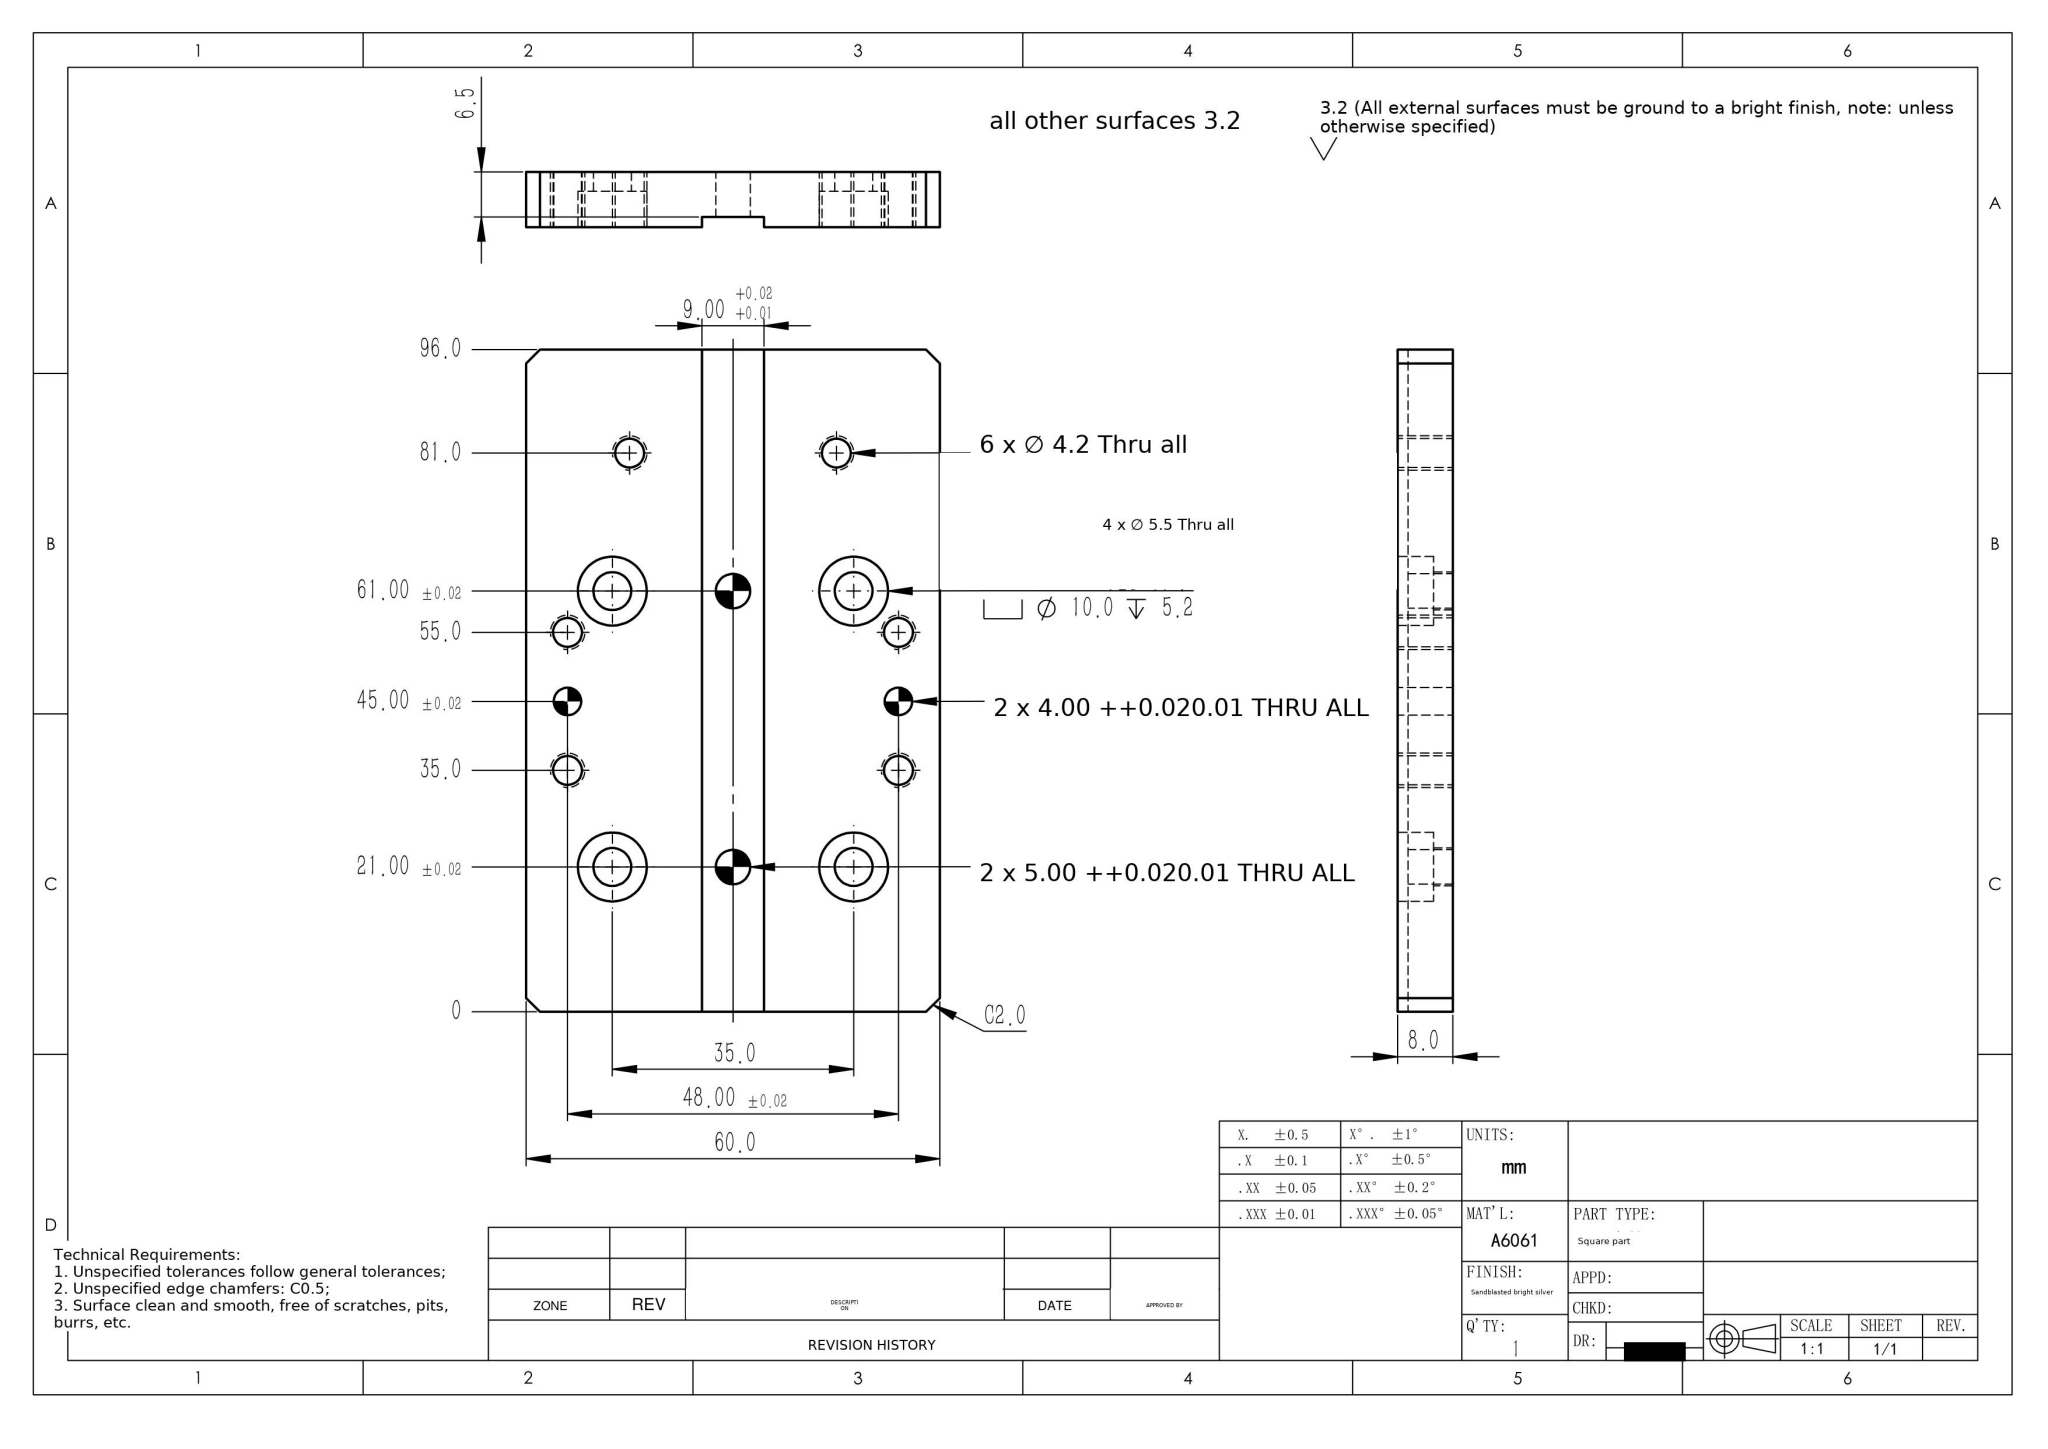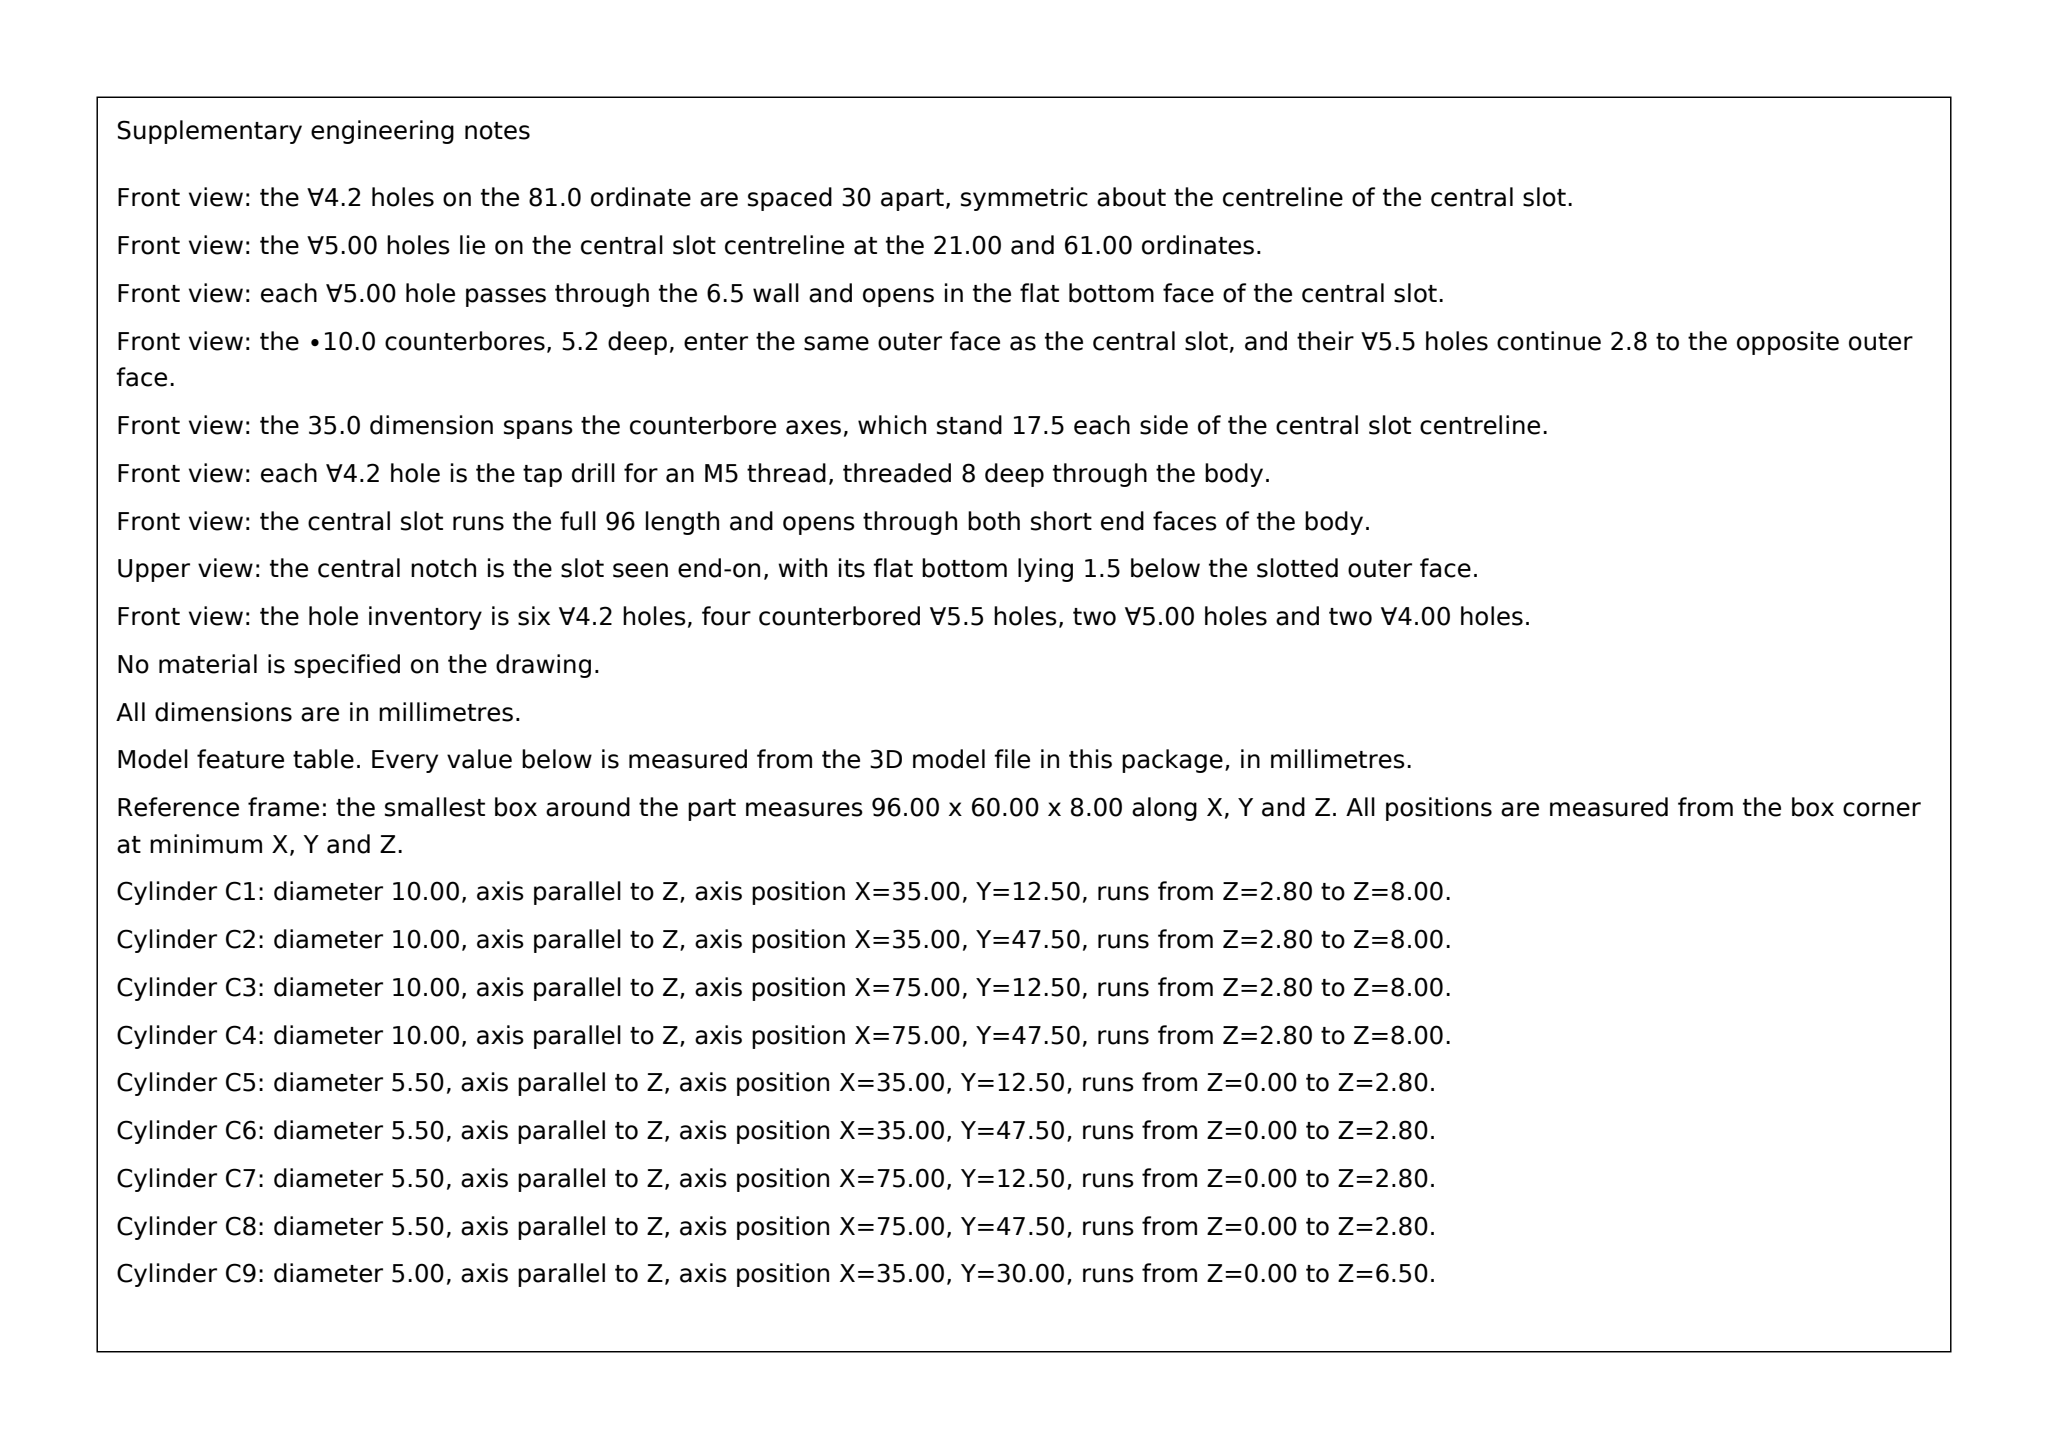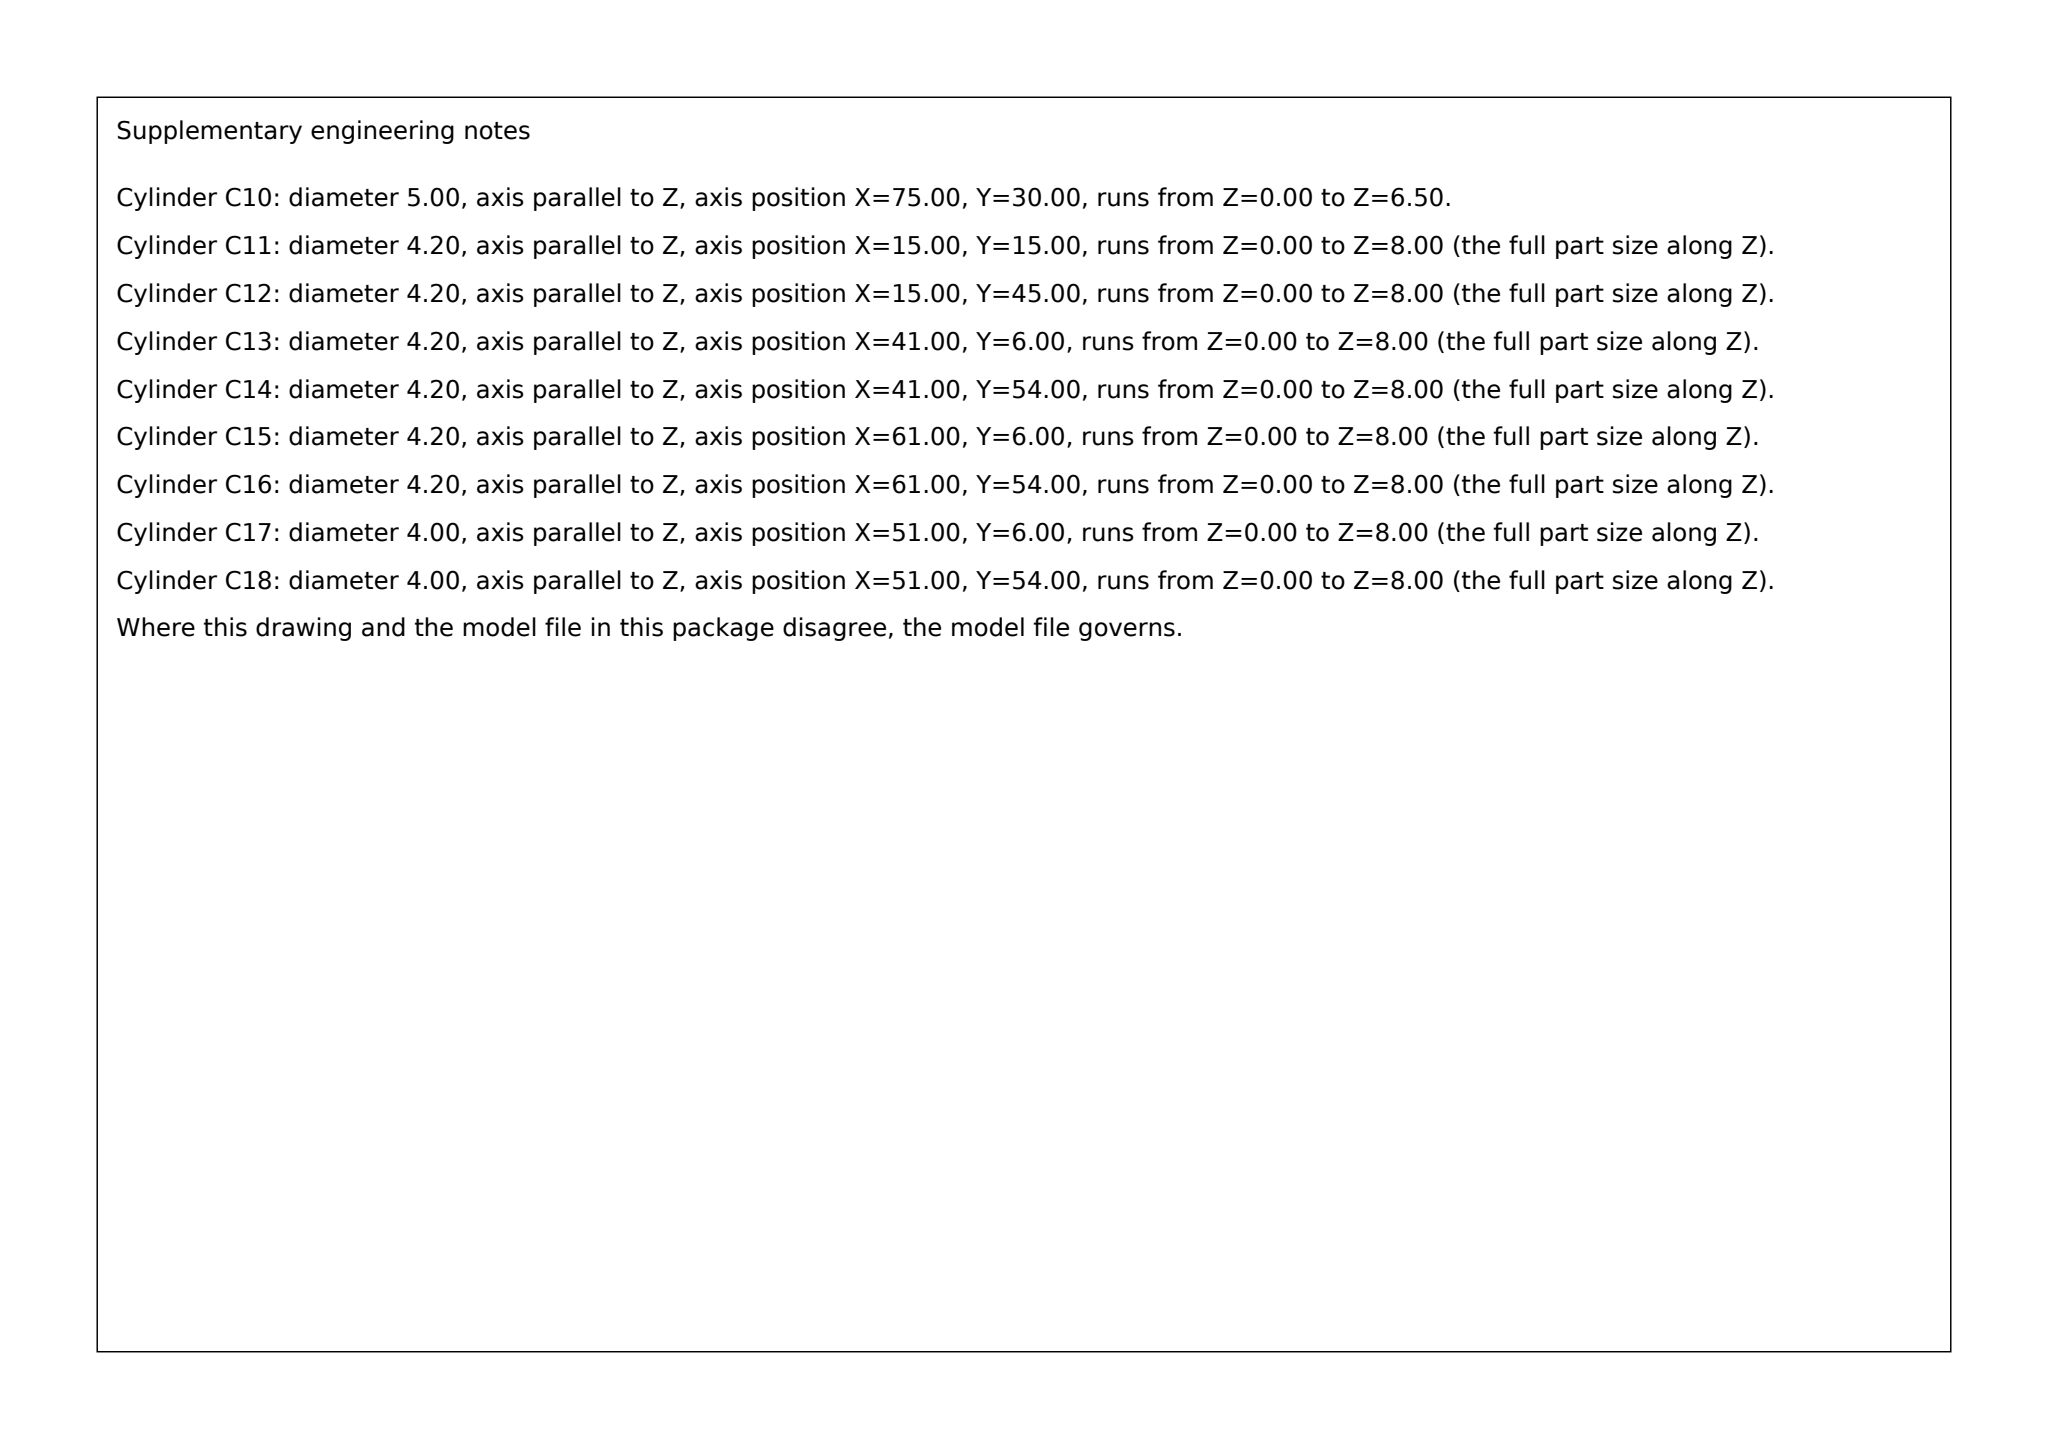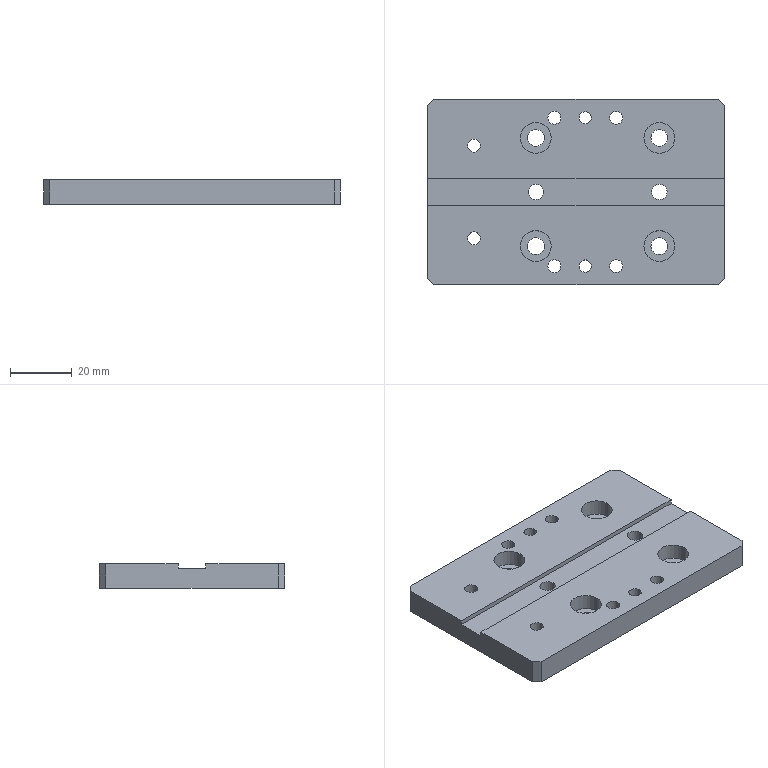Part | SolidWorks | mm | 1 solid | 54 faces | box 96 x 60 x 8 mm | volume 41699 mm3 | cylinder 36 | plane 18 | commonest cylinder face diameters 4.2 x12 10 x8 5.5 x8 4 x4 5 x4
Drawing notes:
GROOVE 9.00 W X 1.5 DP, FULL 96 LG, SYM ABT CL, FLOOR 6.5 FROM BACK FACE | from the solid: y planes 25.5 & 34.5 (9 wide, ctr y=30); z plane 6.5 vs top 8.0; runs full 96 length
6 X Ø4.2 THRU: TOP PAIR 30.0 APART (15.0 EA SIDE), LWR 4 ON 48.00 CRS, SYM ABT CL | from the solid: Ø4.2 at y=15 & 45 (x=15); Ø4.2 at y=6 & 54 for x=41 and x=61; bbox width 60, CL y=30
4 X Ø5.5 THRU, CBORE Ø10.0 DP 5.2, ON 35.0 CRS, SYM ABT CL | from the solid: Ø5.5/Ø10.0 pairs at y=12.5 & 47.5 (35 apart), x=35 & 75, sym abt y=30
2 X Ø4.00 THRU ON 48.00 CRS, SYM ABT CL, 45.00 FROM BTM EDGE | from the solid: Ø4.0 cyls at (x=51,y=6) & (x=51,y=54); 96-51=45
2 X Ø5.00 THRU ON VERT CL, 30.0 FROM EA SIDE | from the solid: Ø5.0 cyls at y=30, x=35 & 75 (= 61.00 & 21.00 from bottom edge)
build123d program:
from build123d import *

# Parameters (mm, degrees)
SKETCH1_W                                       = 96
SKETCH1_H                                       = 60
BOSS_EXTRUDE1_DEPTH                             = 8
M5_HEX_SOCKET_HEAD_CAP_SCREW_CBORE1_D           = 5.5
M5_HEX_SOCKET_HEAD_CAP_SCREW_CBORE1_CBORE_D     = 10
M5_HEX_SOCKET_HEAD_CAP_SCREW_CBORE1_CBORE_DEPTH = 5.2
SIZE_MM_DOWEL_PIN_HOLE1_D                       = 5
M5_TAPPED_HOLE1_D                               = 4.2
SIZE_MM_DOWEL_PIN_HOLE2_D                       = 4
SKETCH10_W                                      = 96
SKETCH10_H                                      = 9
CUT_EXTRUDE1_DEPTH                              = 1.5
CHAMFER1_SIZE                                   = 2


with BuildPart() as part:
    # Sketch1 → Boss-Extrude1 (new body)
    with BuildSketch(Plane.XY):
        Rectangle(SKETCH1_W, SKETCH1_H)
    extrude(amount=BOSS_EXTRUDE1_DEPTH)

    # M5 Hex Socket Head Cap Screw CBORE1 (through all)
    with Locations(Plane.XY.offset(8)):
        with Locations((27, -17.5), (27, 17.5), (-13, 17.5), (-13, -17.5)):
            CounterBoreHole(M5_HEX_SOCKET_HEAD_CAP_SCREW_CBORE1_D / 2, M5_HEX_SOCKET_HEAD_CAP_SCREW_CBORE1_CBORE_D / 2, M5_HEX_SOCKET_HEAD_CAP_SCREW_CBORE1_CBORE_DEPTH)

    # Size mm Dowel Pin Hole1 (through all)
    with Locations(Plane.XY.offset(8)):
        with Locations((27, 0), (-13, 0)):
            Hole(SIZE_MM_DOWEL_PIN_HOLE1_D / 2)

    # M5 Tapped Hole1 (through all)
    with Locations(Plane.XY.offset(8)):
        with Locations((13, -24), (-7, -24), (-7, 24), (13, 24), (-33, -15), (-33, 15)):
            Hole(M5_TAPPED_HOLE1_D / 2)

    # Size mm Dowel Pin Hole2 (through all)
    with Locations(Plane.XY.offset(8)):
        with Locations((3, -24), (3, 24)):
            Hole(SIZE_MM_DOWEL_PIN_HOLE2_D / 2)

    # Sketch10 → Cut-Extrude1 (cut)
    with BuildSketch(Plane.XY.offset(8)):
        Rectangle(SKETCH10_W, SKETCH10_H)
    extrude(amount=-CUT_EXTRUDE1_DEPTH, mode=Mode.SUBTRACT)

    # Chamfer1
    chamfer1_edges = [part.edges().sort_by_distance(p)[0] for p in [
        (48, -30, 4),
        (-48, -30, 4),
        (-48, 30, 4),
        (48, 30, 4),
    ]]
    chamfer(chamfer1_edges, length=CHAMFER1_SIZE)


solid = part.part